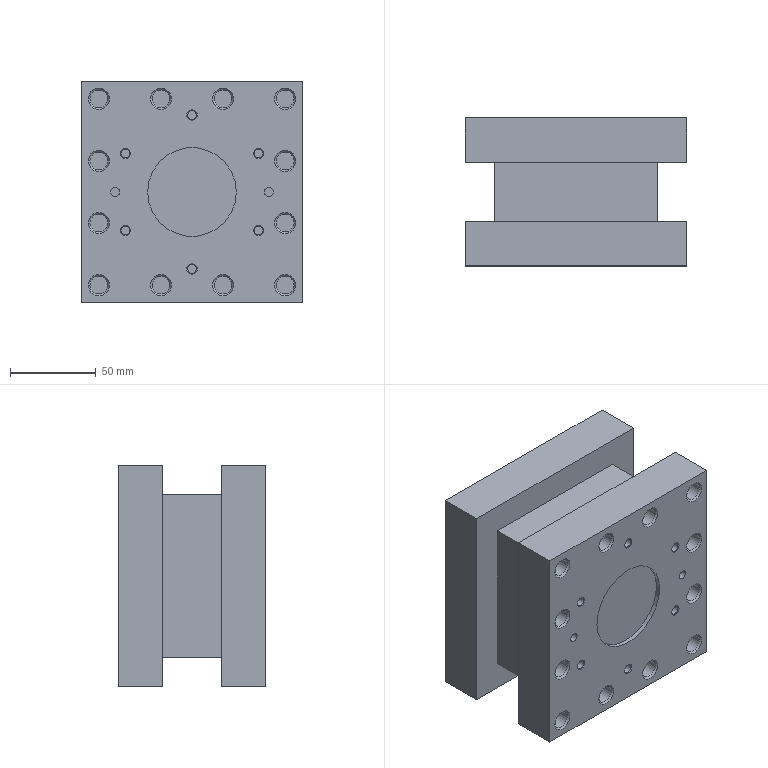Component | NX | TOOL_HOLDER_BODY | 1 solid | 66 faces | volume 1071899 mm3 | plane 26 | cylinder 22 | cone 18 | commonest cylinder face diameters 10.32 x12 5.16 x8 51.6 x1 48 x1